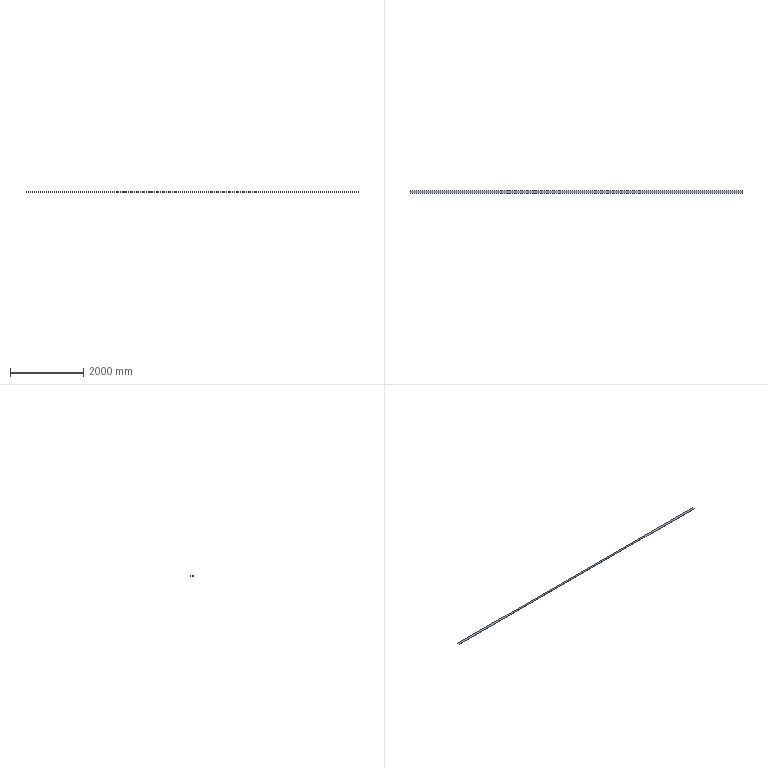Component | SolidWorks | Main-1_9340X60X6-1 | 1 solid | 6 faces | box 9070 x 60 x 6 mm | volume 3265200 mm3 | plane 6 | material Plain Carbon Steel
STEP:
#1=COLOUR_RGB('',0.7922,0.8196,0.9333);
#2=FILL_AREA_STYLE_COLOUR('',#1);
#3=FILL_AREA_STYLE('',(#2));
#4=SURFACE_STYLE_FILL_AREA(#3);
#5=SURFACE_SIDE_STYLE('',(#4));
#6=SURFACE_STYLE_USAGE(.BOTH.,#5);
#7=PRESENTATION_STYLE_ASSIGNMENT((#6));
#8=CARTESIAN_POINT('',(-120.953,83.28,204.408));
#9=VERTEX_POINT('',#8);
#10=CARTESIAN_POINT('',(-120.953,80.918,204.408));
#11=VERTEX_POINT('',#10);
#12=CARTESIAN_POINT('',(-120.953,83.28,204.408));
#13=DIRECTION('',(0.,-1.,-0.));
#14=VECTOR('',#13,39.37);
#15=LINE('',#12,#14);
#16=EDGE_CURVE('',#9,#11,#15,.T.);
#17=ORIENTED_EDGE('',*,*,#16,.F.);
#18=CARTESIAN_POINT('',(-120.953,83.28,204.172));
#19=VERTEX_POINT('',#18);
#20=CARTESIAN_POINT('',(-120.953,83.28,204.172));
#21=DIRECTION('',(0.,-0.,1.));
#22=VECTOR('',#21,39.37);
#23=LINE('',#20,#22);
#24=EDGE_CURVE('',#19,#9,#23,.T.);
#25=ORIENTED_EDGE('',*,*,#24,.F.);
#26=CARTESIAN_POINT('',(-120.953,80.918,204.172));
#27=VERTEX_POINT('',#26);
#28=CARTESIAN_POINT('',(-120.953,83.28,204.172));
#29=DIRECTION('',(0.,-1.,-0.));
#30=VECTOR('',#29,39.37);
#31=LINE('',#28,#30);
#32=EDGE_CURVE('',#19,#27,#31,.T.);
#33=ORIENTED_EDGE('',*,*,#32,.T.);
#34=CARTESIAN_POINT('',(-120.953,80.918,204.172));
#35=DIRECTION('',(0.,-0.,1.));
#36=VECTOR('',#35,39.37);
#37=LINE('',#34,#36);
#38=EDGE_CURVE('',#27,#11,#37,.T.);
#39=ORIENTED_EDGE('',*,*,#38,.T.);
#40=EDGE_LOOP('',(#17,#25,#33,#39));
#41=FACE_OUTER_BOUND('',#40,.T.);
#42=CARTESIAN_POINT('',(-120.953,83.28,204.172));
#43=DIRECTION('',(-1.,-0.,-0.));
#44=DIRECTION('',(0.,-1.,-0.));
#45=AXIS2_PLACEMENT_3D('',#42,#43,#44);
#46=PLANE('',#45);
#47=ADVANCED_FACE('',(#41),#46,.T.);
#48=CARTESIAN_POINT('',(236.134,83.28,204.408));
#49=VERTEX_POINT('',#48);
#50=CARTESIAN_POINT('',(-120.953,83.28,204.408));
#51=DIRECTION('',(-1.,0.,0.));
#52=VECTOR('',#51,39.37);
#53=LINE('',#50,#52);
#54=EDGE_CURVE('',#49,#9,#53,.T.);
#55=ORIENTED_EDGE('',*,*,#54,.F.);
#56=CARTESIAN_POINT('',(236.134,83.28,204.172));
#57=VERTEX_POINT('',#56);
#58=CARTESIAN_POINT('',(236.134,83.28,204.172));
#59=DIRECTION('',(0.,-0.,1.));
#60=VECTOR('',#59,39.37);
#61=LINE('',#58,#60);
#62=EDGE_CURVE('',#57,#49,#61,.T.);
#63=ORIENTED_EDGE('',*,*,#62,.F.);
#64=CARTESIAN_POINT('',(-120.953,83.28,204.172));
#65=DIRECTION('',(-1.,0.,0.));
#66=VECTOR('',#65,39.37);
#67=LINE('',#64,#66);
#68=EDGE_CURVE('',#57,#19,#67,.T.);
#69=ORIENTED_EDGE('',*,*,#68,.T.);
#70=ORIENTED_EDGE('',*,*,#24,.T.);
#71=EDGE_LOOP('',(#55,#63,#69,#70));
#72=FACE_OUTER_BOUND('',#71,.T.);
#73=CARTESIAN_POINT('',(-120.953,83.28,204.172));
#74=DIRECTION('',(0.,1.,0.));
#75=DIRECTION('',(-1.,0.,0.));
#76=AXIS2_PLACEMENT_3D('',#73,#74,#75);
#77=PLANE('',#76);
#78=ADVANCED_FACE('',(#72),#77,.T.);
#79=CARTESIAN_POINT('',(236.134,80.918,204.408));
#80=VERTEX_POINT('',#79);
#81=CARTESIAN_POINT('',(236.134,83.28,204.408));
#82=DIRECTION('',(0.,1.,0.));
#83=VECTOR('',#82,39.37);
#84=LINE('',#81,#83);
#85=EDGE_CURVE('',#80,#49,#84,.T.);
#86=ORIENTED_EDGE('',*,*,#85,.F.);
#87=CARTESIAN_POINT('',(236.134,80.918,204.172));
#88=VERTEX_POINT('',#87);
#89=CARTESIAN_POINT('',(236.134,80.918,204.172));
#90=DIRECTION('',(0.,-0.,1.));
#91=VECTOR('',#90,39.37);
#92=LINE('',#89,#91);
#93=EDGE_CURVE('',#88,#80,#92,.T.);
#94=ORIENTED_EDGE('',*,*,#93,.F.);
#95=CARTESIAN_POINT('',(236.134,83.28,204.172));
#96=DIRECTION('',(0.,1.,0.));
#97=VECTOR('',#96,39.37);
#98=LINE('',#95,#97);
#99=EDGE_CURVE('',#88,#57,#98,.T.);
#100=ORIENTED_EDGE('',*,*,#99,.T.);
#101=ORIENTED_EDGE('',*,*,#62,.T.);
#102=EDGE_LOOP('',(#86,#94,#100,#101));
#103=FACE_OUTER_BOUND('',#102,.T.);
#104=CARTESIAN_POINT('',(236.134,83.28,204.172));
#105=DIRECTION('',(1.,0.,0.));
#106=DIRECTION('',(0.,1.,0.));
#107=AXIS2_PLACEMENT_3D('',#104,#105,#106);
#108=PLANE('',#107);
#109=ADVANCED_FACE('',(#103),#108,.T.);
#110=CARTESIAN_POINT('',(-120.953,80.918,204.408));
#111=DIRECTION('',(1.,0.,0.));
#112=VECTOR('',#111,39.37);
#113=LINE('',#110,#112);
#114=EDGE_CURVE('',#11,#80,#113,.T.);
#115=ORIENTED_EDGE('',*,*,#114,.F.);
#116=ORIENTED_EDGE('',*,*,#38,.F.);
#117=CARTESIAN_POINT('',(-120.953,80.918,204.172));
#118=DIRECTION('',(1.,0.,0.));
#119=VECTOR('',#118,39.37);
#120=LINE('',#117,#119);
#121=EDGE_CURVE('',#27,#88,#120,.T.);
#122=ORIENTED_EDGE('',*,*,#121,.T.);
#123=ORIENTED_EDGE('',*,*,#93,.T.);
#124=EDGE_LOOP('',(#115,#116,#122,#123));
#125=FACE_OUTER_BOUND('',#124,.T.);
#126=CARTESIAN_POINT('',(-120.953,80.918,204.172));
#127=DIRECTION('',(0.,-1.,-0.));
#128=DIRECTION('',(1.,0.,0.));
#129=AXIS2_PLACEMENT_3D('',#126,#127,#128);
#130=PLANE('',#129);
#131=ADVANCED_FACE('',(#125),#130,.T.);
#132=ORIENTED_EDGE('',*,*,#32,.F.);
#133=ORIENTED_EDGE('',*,*,#68,.F.);
#134=ORIENTED_EDGE('',*,*,#99,.F.);
#135=ORIENTED_EDGE('',*,*,#121,.F.);
#136=EDGE_LOOP('',(#132,#133,#134,#135));
#137=FACE_OUTER_BOUND('',#136,.T.);
#138=CARTESIAN_POINT('',(-120.953,83.28,204.172));
#139=DIRECTION('',(0.,-0.,1.));
#140=DIRECTION('',(0.,-1.,-0.));
#141=AXIS2_PLACEMENT_3D('',#138,#139,#140);
#142=PLANE('',#141);
#143=ADVANCED_FACE('',(#137),#142,.F.);
#144=ORIENTED_EDGE('',*,*,#16,.T.);
#145=ORIENTED_EDGE('',*,*,#114,.T.);
#146=ORIENTED_EDGE('',*,*,#85,.T.);
#147=ORIENTED_EDGE('',*,*,#54,.T.);
#148=EDGE_LOOP('',(#144,#145,#146,#147));
#149=FACE_OUTER_BOUND('',#148,.T.);
#150=CARTESIAN_POINT('',(-120.953,83.28,204.408));
#151=DIRECTION('',(0.,-0.,1.));
#152=DIRECTION('',(0.,-1.,-0.));
#153=AXIS2_PLACEMENT_3D('',#150,#151,#152);
#154=PLANE('',#153);
#155=ADVANCED_FACE('',(#149),#154,.T.);
#156=CLOSED_SHELL('',(#47,#78,#109,#131,#143,#155));
#157=MANIFOLD_SOLID_BREP('',#156);
#158=STYLED_ITEM('',(#7),#157);
#159=PRESENTATION_LAYER_ASSIGNMENT('','',(#158));
#160=(LENGTH_UNIT()NAMED_UNIT(*)SI_UNIT($,.METRE.));
#161=LENGTH_MEASURE_WITH_UNIT(LENGTH_MEASURE(0.0254),#160);
#162=DIMENSIONAL_EXPONENTS(1.,0.,0.,0.,0.,0.,0.);
#163=(CONVERSION_BASED_UNIT('',#161)LENGTH_UNIT()NAMED_UNIT(#162));
#164=UNCERTAINTY_MEASURE_WITH_UNIT(LENGTH_MEASURE(0.00001),#163,'','');
#165=(NAMED_UNIT(*)PLANE_ANGLE_UNIT()SI_UNIT($,.RADIAN.));
#166=(NAMED_UNIT(*)SI_UNIT($,.STERADIAN.)SOLID_ANGLE_UNIT());
#167=(GEOMETRIC_REPRESENTATION_CONTEXT(3)GLOBAL_UNCERTAINTY_ASSIGNED_CONTEXT((#164))GLOBAL_UNIT_ASSIGNED_CONTEXT((#163,#165,#166))REPRESENTATION_CONTEXT('',''));
#168=MECHANICAL_DESIGN_GEOMETRIC_PRESENTATION_REPRESENTATION('',(#158),#167);
#169=CARTESIAN_POINT('',(0.,0.,0.));
#170=DIRECTION('',(0.,0.,1.));
#171=DIRECTION('',(1.,0.,0.));
#172=AXIS2_PLACEMENT_3D('',#169,#170,#171);
#173=(LENGTH_UNIT()NAMED_UNIT(*)SI_UNIT($,.METRE.));
#174=LENGTH_MEASURE_WITH_UNIT(LENGTH_MEASURE(0.0254),#173);
#175=DIMENSIONAL_EXPONENTS(1.,0.,0.,0.,0.,0.,0.);
#176=(CONVERSION_BASED_UNIT('',#174)LENGTH_UNIT()NAMED_UNIT(#175));
#177=UNCERTAINTY_MEASURE_WITH_UNIT(LENGTH_MEASURE(0.00001),#176,'','');
#178=(NAMED_UNIT(*)PLANE_ANGLE_UNIT()SI_UNIT($,.RADIAN.));
#179=(NAMED_UNIT(*)SI_UNIT($,.STERADIAN.)SOLID_ANGLE_UNIT());
#180=(GEOMETRIC_REPRESENTATION_CONTEXT(3)GLOBAL_UNCERTAINTY_ASSIGNED_CONTEXT((#177))GLOBAL_UNIT_ASSIGNED_CONTEXT((#176,#178,#179))REPRESENTATION_CONTEXT('',''));
#181=ADVANCED_BREP_SHAPE_REPRESENTATION('',(#157,#172),#180);